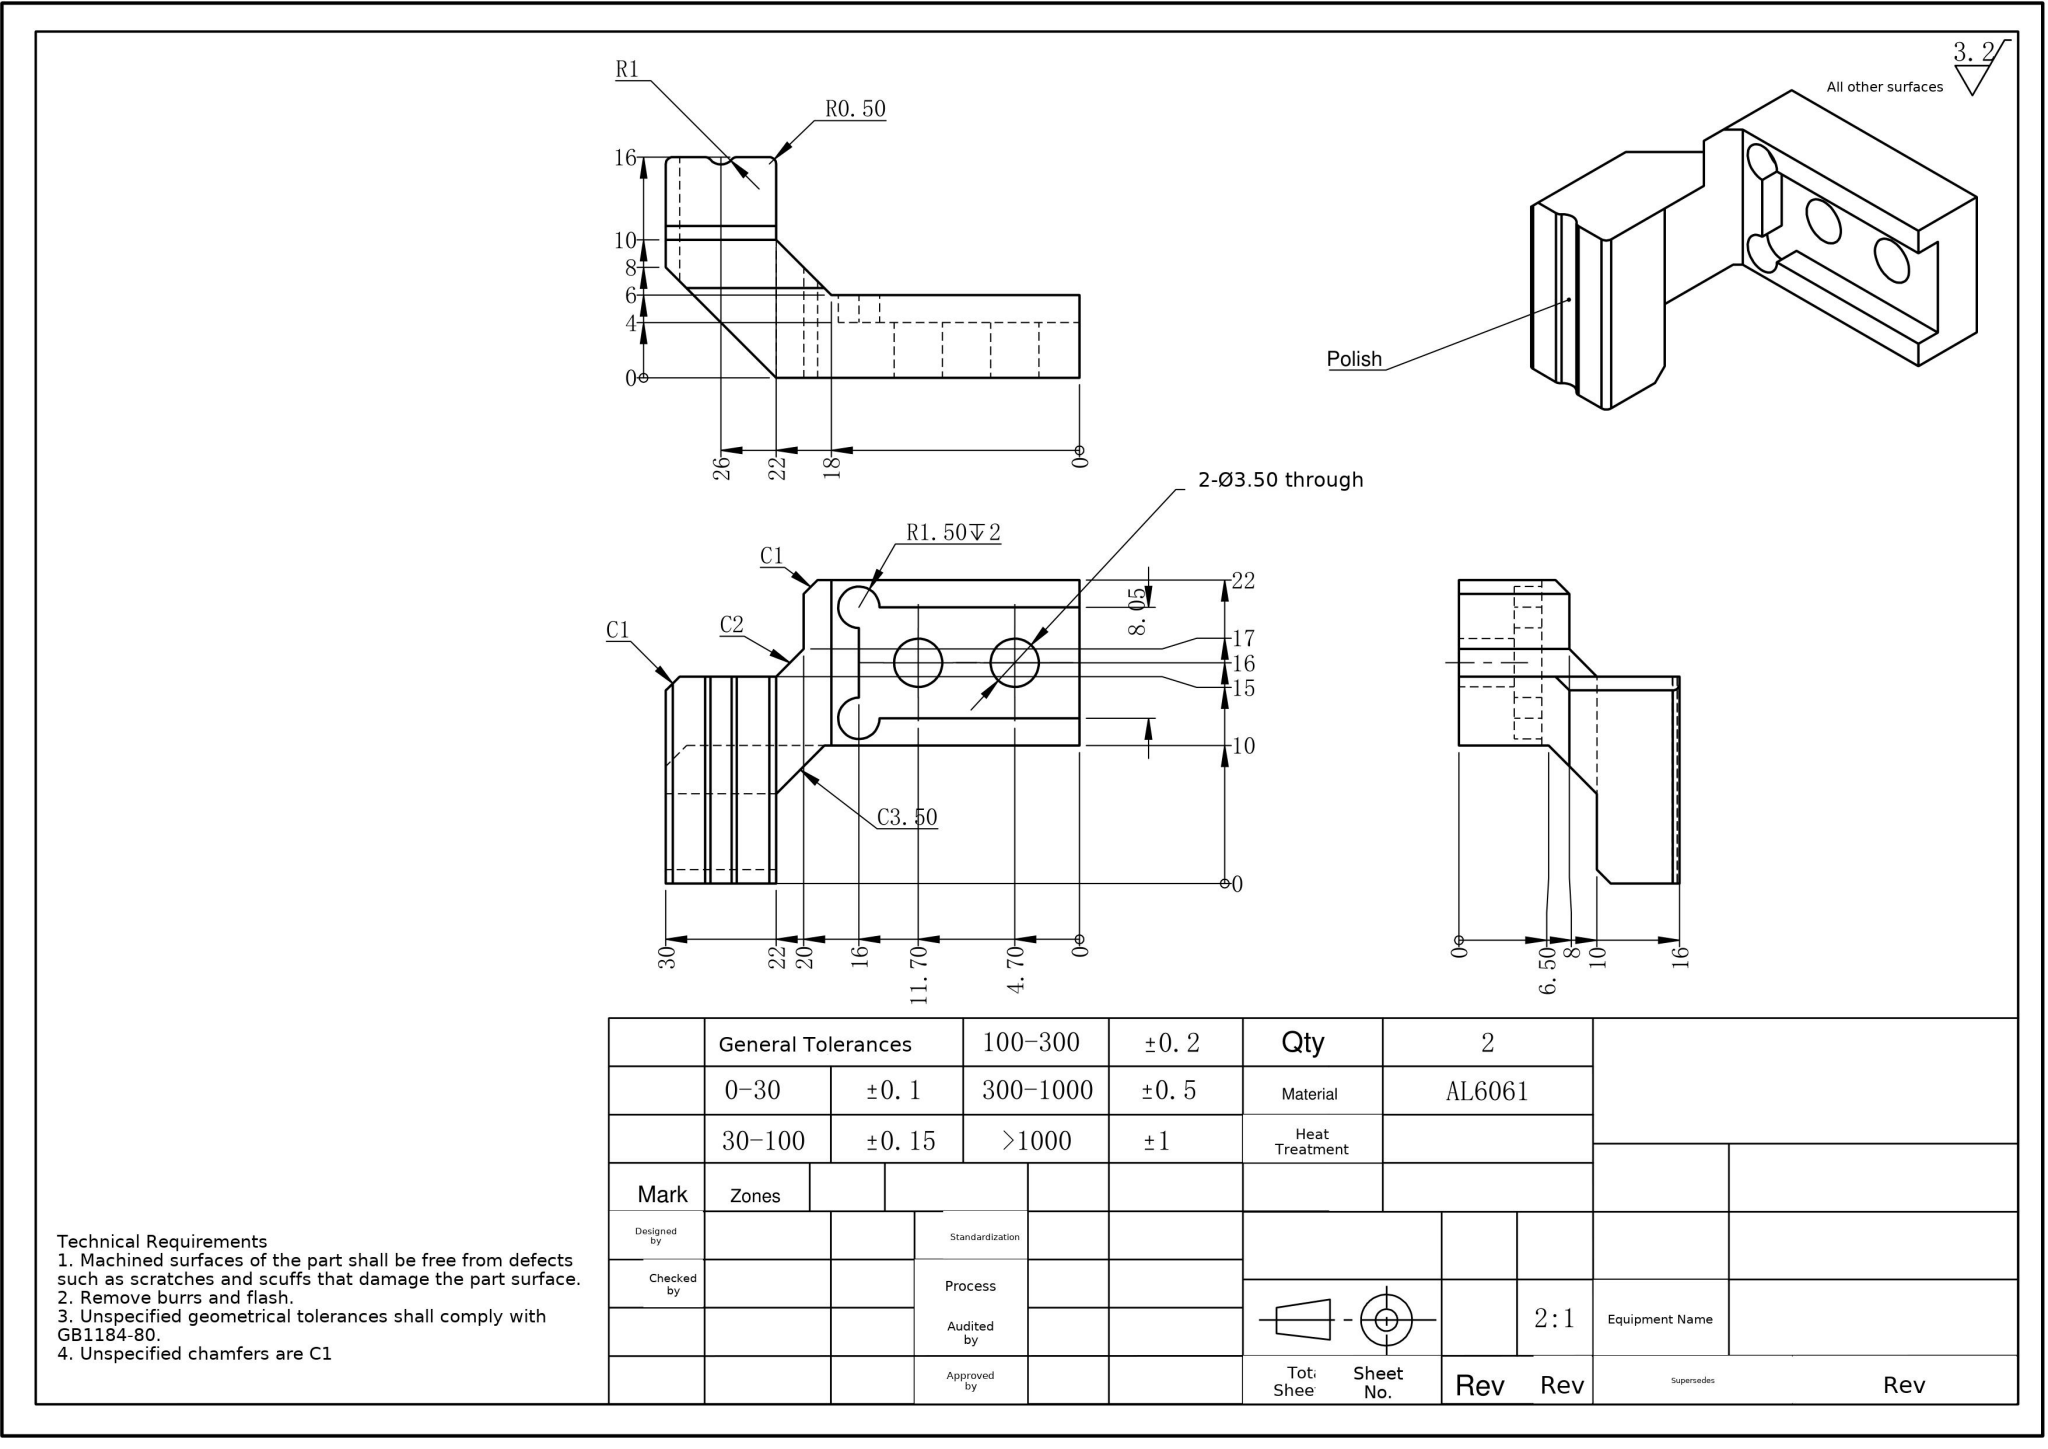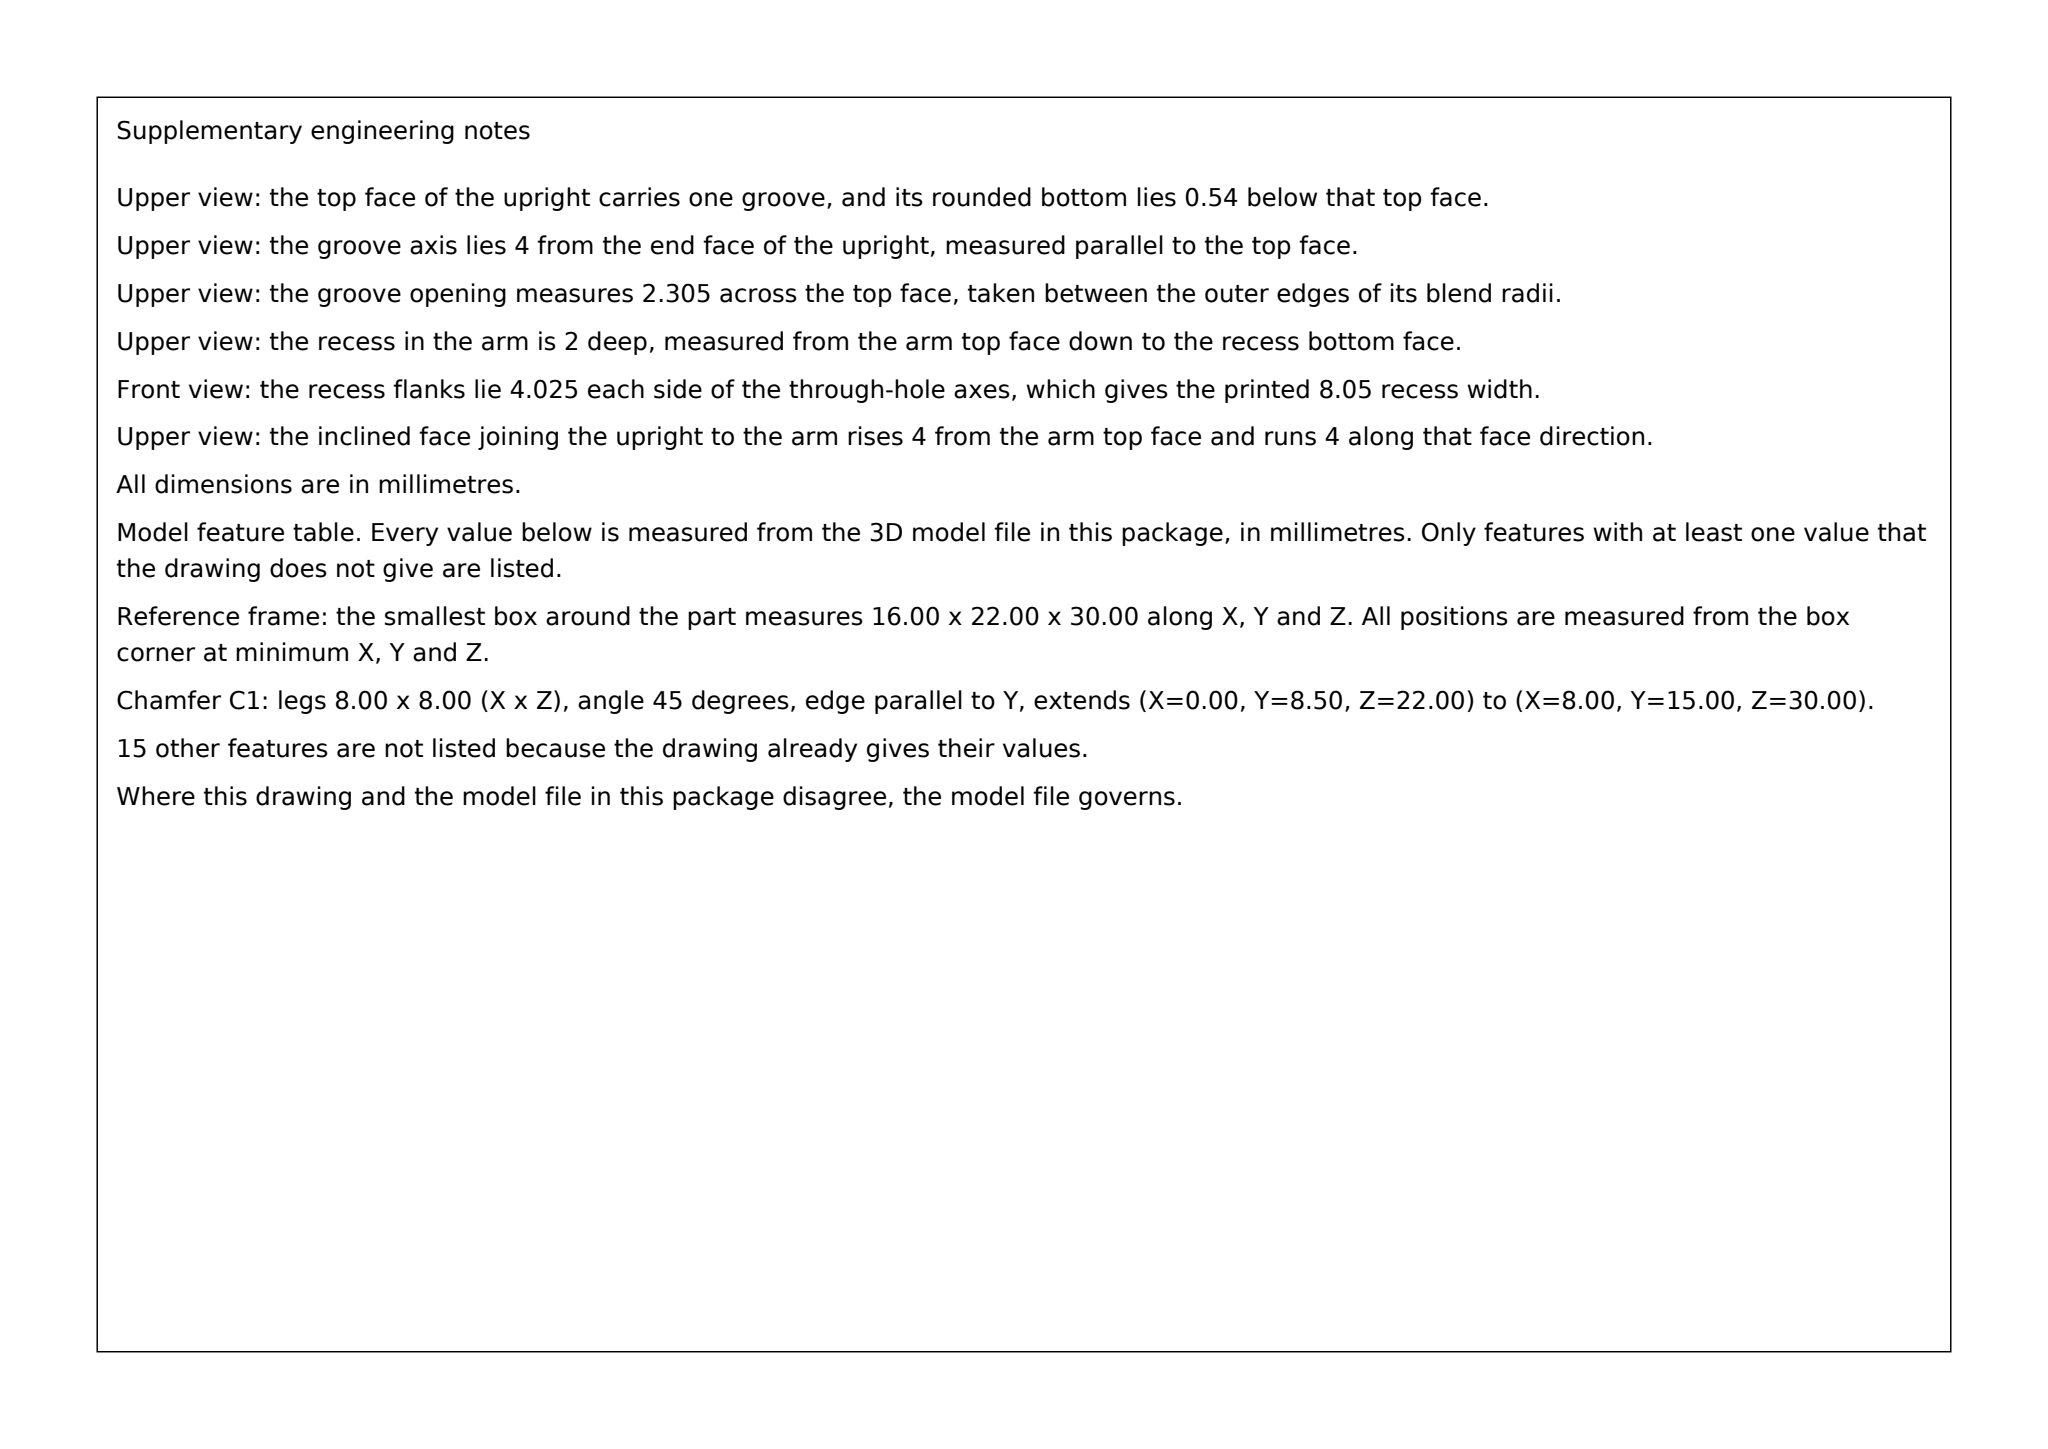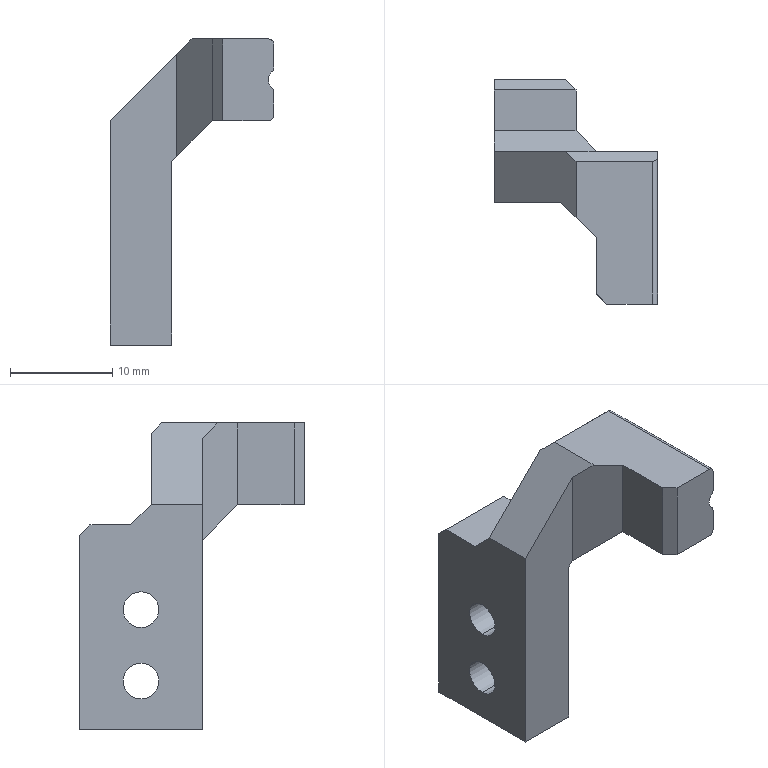Part | SolidWorks | mm | 1 solid | 37 faces | box 16 x 22 x 30 mm | volume 2207 mm3 | plane 24 | cylinder 13 | commonest cylinder face diameters 3.5 x4 3 x4 1 x4 2 x1
Drawing notes:
4 X R0.50 GROOVES ON POLISH FACE AT 22.50, 24.85, 27.15, 29.50 | from the solid: Ø1 y-axis cyls at z=22.5, 24.85, 27.15, 29.5 (x=15.5), from z=0 datum
R0.50 GROOVES 15 LG FROM 0 DATUM; GROOVE AT 29.50 IS 14.5 LG | from the solid: Ø1 cyl lengths 15,15,15 and 14.5 along y, ending at plane y=15
R1 GROOVE DP 0.54 AT 26.00, 15 LG FROM 0 DATUM | from the solid: Ø2 y-axis cyl at x=16.46, z=26.0, len 15; depth 1-(16.46-16)=0.54